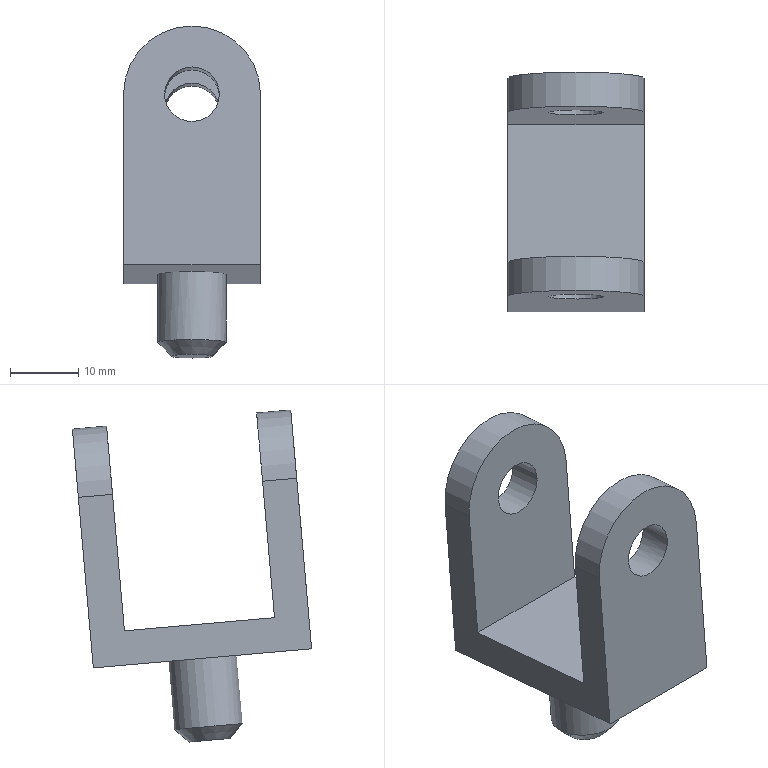Component | NX | LOCATING_SEAT | 1 solid | 15 faces | box 20 x 34.93 x 48.48 mm | volume 9156 mm3 | plane 9 | cylinder 5 | cone 1 | commonest cylinder face diameters 20 x2 8 x2 10 x1
STEP:
#1=CARTESIAN_POINT('',(0.,0.,0.));
#2=DIRECTION('',(0.,0.,1.));
#3=DIRECTION('',(1.,0.,0.));
#4=AXIS2_PLACEMENT_3D('',#1,#2,#3);
#5=CARTESIAN_POINT('',(285.941,457.133,-24.72));
#6=VERTEX_POINT('',#5);
#7=CARTESIAN_POINT('',(265.941,457.133,-24.72));
#8=VERTEX_POINT('',#7);
#9=CARTESIAN_POINT('',(275.941,457.133,-24.72));
#10=DIRECTION('',(0.,-0.9962,0.08716));
#11=DIRECTION('',(-1.,0.,0.));
#12=AXIS2_PLACEMENT_3D('',#9,#10,#11);
#13=CIRCLE('',#12,10.);
#14=CARTESIAN_POINT('',(275.941,462.114,-25.155));
#15=DIRECTION('',(0.,-0.9962,0.08716));
#16=DIRECTION('',(0.,0.08716,0.9962));
#17=AXIS2_PLACEMENT_3D('',#14,#15,#16);
#18=CYLINDRICAL_SURFACE('',#17,10.);
#19=CARTESIAN_POINT('',(-4.712,5.));
#20=DIRECTION('',(1.,0.));
#21=VECTOR('',#20,1.);
#22=LINE('',#19,#21);
#23=(GEOMETRIC_REPRESENTATION_CONTEXT(2)PARAMETRIC_REPRESENTATION_CONTEXT()REPRESENTATION_CONTEXT('',''));
#24=DEFINITIONAL_REPRESENTATION('',(#22),#23);
#25=PCURVE('',#18,#24);
#26=CARTESIAN_POINT('',(275.941,457.133,-24.72));
#27=DIRECTION('',(0.,-0.9962,0.08716));
#28=DIRECTION('',(0.,0.08716,0.9962));
#29=AXIS2_PLACEMENT_3D('',#26,#27,#28);
#30=PLANE('',#29);
#31=CARTESIAN_POINT('',(0.,0.));
#32=DIRECTION('',(0.,1.));
#33=AXIS2_PLACEMENT_2D('',#31,#32);
#34=CIRCLE('',#33,10.);
#35=(GEOMETRIC_REPRESENTATION_CONTEXT(2)PARAMETRIC_REPRESENTATION_CONTEXT()REPRESENTATION_CONTEXT('',''));
#36=DEFINITIONAL_REPRESENTATION('',(#34),#35);
#37=PCURVE('',#30,#36);
#38=SURFACE_CURVE('',#13,(#25,#37),.PCURVE_S1.);
#39=EDGE_CURVE('',#6,#8,#38,.T.);
#40=ORIENTED_EDGE('',*,*,#39,.F.);
#41=CARTESIAN_POINT('',(285.941,462.114,-25.155));
#42=VERTEX_POINT('',#41);
#43=CARTESIAN_POINT('',(285.941,462.114,-25.155));
#44=DIRECTION('',(0.,-0.9962,0.08716));
#45=VECTOR('',#44,1.);
#46=LINE('',#43,#45);
#47=CARTESIAN_POINT('',(-1.571,0.));
#48=DIRECTION('',(0.,1.));
#49=VECTOR('',#48,1.);
#50=LINE('',#47,#49);
#51=(GEOMETRIC_REPRESENTATION_CONTEXT(2)PARAMETRIC_REPRESENTATION_CONTEXT()REPRESENTATION_CONTEXT('',''));
#52=DEFINITIONAL_REPRESENTATION('',(#50),#51);
#53=PCURVE('',#18,#52);
#54=CARTESIAN_POINT('',(285.941,462.114,-25.155));
#55=DIRECTION('',(-1.,0.,0.));
#56=DIRECTION('',(0.,0.08716,0.9962));
#57=AXIS2_PLACEMENT_3D('',#54,#55,#56);
#58=PLANE('',#57);
#59=CARTESIAN_POINT('',(0.,0.));
#60=DIRECTION('',(-0.,-1.));
#61=VECTOR('',#60,1.);
#62=LINE('',#59,#61);
#63=(GEOMETRIC_REPRESENTATION_CONTEXT(2)PARAMETRIC_REPRESENTATION_CONTEXT()REPRESENTATION_CONTEXT('',''));
#64=DEFINITIONAL_REPRESENTATION('',(#62),#63);
#65=PCURVE('',#58,#64);
#66=SURFACE_CURVE('',#46,(#53,#65),.PCURVE_S1.);
#67=EDGE_CURVE('',#42,#6,#66,.T.);
#68=ORIENTED_EDGE('',*,*,#67,.F.);
#69=CARTESIAN_POINT('',(265.941,462.114,-25.155));
#70=VERTEX_POINT('',#69);
#71=CARTESIAN_POINT('',(275.941,462.114,-25.155));
#72=DIRECTION('',(0.,0.9962,-0.08716));
#73=DIRECTION('',(-1.,0.,0.));
#74=AXIS2_PLACEMENT_3D('',#71,#72,#73);
#75=CIRCLE('',#74,10.);
#76=CARTESIAN_POINT('',(1.571,0.));
#77=DIRECTION('',(-1.,0.));
#78=VECTOR('',#77,1.);
#79=LINE('',#76,#78);
#80=(GEOMETRIC_REPRESENTATION_CONTEXT(2)PARAMETRIC_REPRESENTATION_CONTEXT()REPRESENTATION_CONTEXT('',''));
#81=DEFINITIONAL_REPRESENTATION('',(#79),#80);
#82=PCURVE('',#18,#81);
#83=CARTESIAN_POINT('',(275.941,462.114,-25.155));
#84=DIRECTION('',(0.,0.9962,-0.08716));
#85=DIRECTION('',(0.,-0.08716,-0.9962));
#86=AXIS2_PLACEMENT_3D('',#83,#84,#85);
#87=PLANE('',#86);
#88=CARTESIAN_POINT('',(0.,0.));
#89=DIRECTION('',(0.,1.));
#90=AXIS2_PLACEMENT_2D('',#88,#89);
#91=CIRCLE('',#90,10.);
#92=(GEOMETRIC_REPRESENTATION_CONTEXT(2)PARAMETRIC_REPRESENTATION_CONTEXT()REPRESENTATION_CONTEXT('',''));
#93=DEFINITIONAL_REPRESENTATION('',(#91),#92);
#94=PCURVE('',#87,#93);
#95=SURFACE_CURVE('',#75,(#82,#94),.PCURVE_S1.);
#96=EDGE_CURVE('',#70,#42,#95,.T.);
#97=ORIENTED_EDGE('',*,*,#96,.F.);
#98=CARTESIAN_POINT('',(265.941,462.114,-25.155));
#99=DIRECTION('',(0.,-0.9962,0.08716));
#100=VECTOR('',#99,1.);
#101=LINE('',#98,#100);
#102=CARTESIAN_POINT('',(1.571,0.));
#103=DIRECTION('',(0.,1.));
#104=VECTOR('',#103,1.);
#105=LINE('',#102,#104);
#106=(GEOMETRIC_REPRESENTATION_CONTEXT(2)PARAMETRIC_REPRESENTATION_CONTEXT()REPRESENTATION_CONTEXT('',''));
#107=DEFINITIONAL_REPRESENTATION('',(#105),#106);
#108=PCURVE('',#18,#107);
#109=CARTESIAN_POINT('',(265.941,459.935,-50.06));
#110=DIRECTION('',(1.,-0.,-0.));
#111=DIRECTION('',(-0.,-0.08716,-0.9962));
#112=AXIS2_PLACEMENT_3D('',#109,#110,#111);
#113=PLANE('',#112);
#114=CARTESIAN_POINT('',(-25.,-0.));
#115=DIRECTION('',(0.,-1.));
#116=VECTOR('',#115,1.);
#117=LINE('',#114,#116);
#118=(GEOMETRIC_REPRESENTATION_CONTEXT(2)PARAMETRIC_REPRESENTATION_CONTEXT()REPRESENTATION_CONTEXT('',''));
#119=DEFINITIONAL_REPRESENTATION('',(#117),#118);
#120=PCURVE('',#113,#119);
#121=SURFACE_CURVE('',#101,(#108,#120),.PCURVE_S1.);
#122=EDGE_CURVE('',#70,#8,#121,.T.);
#123=ORIENTED_EDGE('',*,*,#122,.T.);
#124=EDGE_LOOP('',(#40,#68,#97,#123));
#125=FACE_BOUND('',#124,.T.);
#126=ADVANCED_FACE('',(#125),#18,.T.);
#127=CARTESIAN_POINT('',(285.941,455.39,-44.644));
#128=VERTEX_POINT('',#127);
#129=CARTESIAN_POINT('',(285.941,433.473,-42.726));
#130=VERTEX_POINT('',#129);
#131=CARTESIAN_POINT('',(285.941,455.39,-44.644));
#132=DIRECTION('',(0.,-0.9962,0.08716));
#133=VECTOR('',#132,1.);
#134=LINE('',#131,#133);
#135=CARTESIAN_POINT('',(-20.,-5.));
#136=DIRECTION('',(-0.,-1.));
#137=VECTOR('',#136,1.);
#138=LINE('',#135,#137);
#139=(GEOMETRIC_REPRESENTATION_CONTEXT(2)PARAMETRIC_REPRESENTATION_CONTEXT()REPRESENTATION_CONTEXT('',''));
#140=DEFINITIONAL_REPRESENTATION('',(#138),#139);
#141=PCURVE('',#58,#140);
#142=CARTESIAN_POINT('',(265.941,455.39,-44.644));
#143=DIRECTION('',(0.,-0.08716,-0.9962));
#144=DIRECTION('',(0.,-0.9962,0.08716));
#145=AXIS2_PLACEMENT_3D('',#142,#143,#144);
#146=PLANE('',#145);
#147=CARTESIAN_POINT('',(0.,-20.));
#148=DIRECTION('',(1.,0.));
#149=VECTOR('',#148,1.);
#150=LINE('',#147,#149);
#151=(GEOMETRIC_REPRESENTATION_CONTEXT(2)PARAMETRIC_REPRESENTATION_CONTEXT()REPRESENTATION_CONTEXT('',''));
#152=DEFINITIONAL_REPRESENTATION('',(#150),#151);
#153=PCURVE('',#146,#152);
#154=SURFACE_CURVE('',#134,(#141,#153),.PCURVE_S1.);
#155=EDGE_CURVE('',#128,#130,#154,.T.);
#156=ORIENTED_EDGE('',*,*,#155,.T.);
#157=CARTESIAN_POINT('',(285.941,435.216,-22.802));
#158=VERTEX_POINT('',#157);
#159=CARTESIAN_POINT('',(285.941,433.473,-42.726));
#160=DIRECTION('',(0.,0.08716,0.9962));
#161=VECTOR('',#160,1.);
#162=LINE('',#159,#161);
#163=CARTESIAN_POINT('',(-20.,-27.));
#164=DIRECTION('',(1.,0.));
#165=VECTOR('',#164,1.);
#166=LINE('',#163,#165);
#167=(GEOMETRIC_REPRESENTATION_CONTEXT(2)PARAMETRIC_REPRESENTATION_CONTEXT()REPRESENTATION_CONTEXT('',''));
#168=DEFINITIONAL_REPRESENTATION('',(#166),#167);
#169=PCURVE('',#58,#168);
#170=CARTESIAN_POINT('',(275.941,435.216,-22.802));
#171=DIRECTION('',(0.,-0.9962,0.08716));
#172=DIRECTION('',(0.,0.08716,0.9962));
#173=AXIS2_PLACEMENT_3D('',#170,#171,#172);
#174=PLANE('',#173);
#175=CARTESIAN_POINT('',(-20.,-10.));
#176=DIRECTION('',(1.,-0.));
#177=VECTOR('',#176,1.);
#178=LINE('',#175,#177);
#179=(GEOMETRIC_REPRESENTATION_CONTEXT(2)PARAMETRIC_REPRESENTATION_CONTEXT()REPRESENTATION_CONTEXT('',''));
#180=DEFINITIONAL_REPRESENTATION('',(#178),#179);
#181=PCURVE('',#174,#180);
#182=SURFACE_CURVE('',#162,(#169,#181),.PCURVE_S1.);
#183=EDGE_CURVE('',#130,#158,#182,.T.);
#184=ORIENTED_EDGE('',*,*,#183,.T.);
#185=CARTESIAN_POINT('',(285.941,430.235,-22.367));
#186=VERTEX_POINT('',#185);
#187=CARTESIAN_POINT('',(285.941,462.114,-25.155));
#188=DIRECTION('',(0.,-0.9962,0.08716));
#189=VECTOR('',#188,1.);
#190=LINE('',#187,#189);
#191=CARTESIAN_POINT('',(0.,0.));
#192=DIRECTION('',(-0.,-1.));
#193=VECTOR('',#192,1.);
#194=LINE('',#191,#193);
#195=(GEOMETRIC_REPRESENTATION_CONTEXT(2)PARAMETRIC_REPRESENTATION_CONTEXT()REPRESENTATION_CONTEXT('',''));
#196=DEFINITIONAL_REPRESENTATION('',(#194),#195);
#197=PCURVE('',#58,#196);
#198=CARTESIAN_POINT('',(275.941,462.114,-25.155));
#199=DIRECTION('',(0.,-0.9962,0.08716));
#200=DIRECTION('',(0.,0.08716,0.9962));
#201=AXIS2_PLACEMENT_3D('',#198,#199,#200);
#202=CYLINDRICAL_SURFACE('',#201,10.);
#203=CARTESIAN_POINT('',(4.712,0.));
#204=DIRECTION('',(0.,1.));
#205=VECTOR('',#204,1.);
#206=LINE('',#203,#205);
#207=(GEOMETRIC_REPRESENTATION_CONTEXT(2)PARAMETRIC_REPRESENTATION_CONTEXT()REPRESENTATION_CONTEXT('',''));
#208=DEFINITIONAL_REPRESENTATION('',(#206),#207);
#209=PCURVE('',#202,#208);
#210=SURFACE_CURVE('',#190,(#197,#209),.PCURVE_S1.);
#211=EDGE_CURVE('',#158,#186,#210,.T.);
#212=ORIENTED_EDGE('',*,*,#211,.T.);
#213=CARTESIAN_POINT('',(285.941,428.057,-47.271));
#214=VERTEX_POINT('',#213);
#215=CARTESIAN_POINT('',(285.941,430.235,-22.367));
#216=DIRECTION('',(-0.,-0.08716,-0.9962));
#217=VECTOR('',#216,1.);
#218=LINE('',#215,#217);
#219=CARTESIAN_POINT('',(0.,-32.));
#220=DIRECTION('',(-1.,0.));
#221=VECTOR('',#220,1.);
#222=LINE('',#219,#221);
#223=(GEOMETRIC_REPRESENTATION_CONTEXT(2)PARAMETRIC_REPRESENTATION_CONTEXT()REPRESENTATION_CONTEXT('',''));
#224=DEFINITIONAL_REPRESENTATION('',(#222),#223);
#225=PCURVE('',#58,#224);
#226=CARTESIAN_POINT('',(275.941,430.235,-22.367));
#227=DIRECTION('',(0.,0.9962,-0.08716));
#228=DIRECTION('',(0.,-0.08716,-0.9962));
#229=AXIS2_PLACEMENT_3D('',#226,#227,#228);
#230=PLANE('',#229);
#231=CARTESIAN_POINT('',(0.,-10.));
#232=DIRECTION('',(1.,0.));
#233=VECTOR('',#232,1.);
#234=LINE('',#231,#233);
#235=(GEOMETRIC_REPRESENTATION_CONTEXT(2)PARAMETRIC_REPRESENTATION_CONTEXT()REPRESENTATION_CONTEXT('',''));
#236=DEFINITIONAL_REPRESENTATION('',(#234),#235);
#237=PCURVE('',#230,#236);
#238=SURFACE_CURVE('',#218,(#225,#237),.PCURVE_S1.);
#239=EDGE_CURVE('',#186,#214,#238,.T.);
#240=ORIENTED_EDGE('',*,*,#239,.T.);
#241=CARTESIAN_POINT('',(285.941,459.935,-50.06));
#242=VERTEX_POINT('',#241);
#243=CARTESIAN_POINT('',(285.941,459.935,-50.06));
#244=DIRECTION('',(0.,-0.9962,0.08716));
#245=VECTOR('',#244,1.);
#246=LINE('',#243,#245);
#247=CARTESIAN_POINT('',(-25.,0.));
#248=DIRECTION('',(-0.,-1.));
#249=VECTOR('',#248,1.);
#250=LINE('',#247,#249);
#251=(GEOMETRIC_REPRESENTATION_CONTEXT(2)PARAMETRIC_REPRESENTATION_CONTEXT()REPRESENTATION_CONTEXT('',''));
#252=DEFINITIONAL_REPRESENTATION('',(#250),#251);
#253=PCURVE('',#58,#252);
#254=CARTESIAN_POINT('',(275.941,459.935,-50.06));
#255=DIRECTION('',(0.,0.08716,0.9962));
#256=DIRECTION('',(0.,0.9962,-0.08716));
#257=AXIS2_PLACEMENT_3D('',#254,#255,#256);
#258=PLANE('',#257);
#259=CARTESIAN_POINT('',(0.,-10.));
#260=DIRECTION('',(-1.,0.));
#261=VECTOR('',#260,1.);
#262=LINE('',#259,#261);
#263=(GEOMETRIC_REPRESENTATION_CONTEXT(2)PARAMETRIC_REPRESENTATION_CONTEXT()REPRESENTATION_CONTEXT('',''));
#264=DEFINITIONAL_REPRESENTATION('',(#262),#263);
#265=PCURVE('',#258,#264);
#266=SURFACE_CURVE('',#246,(#253,#265),.PCURVE_S1.);
#267=EDGE_CURVE('',#242,#214,#266,.T.);
#268=ORIENTED_EDGE('',*,*,#267,.F.);
#269=CARTESIAN_POINT('',(285.941,462.114,-25.155));
#270=DIRECTION('',(-0.,-0.08716,-0.9962));
#271=VECTOR('',#270,1.);
#272=LINE('',#269,#271);
#273=CARTESIAN_POINT('',(0.,0.));
#274=DIRECTION('',(-1.,0.));
#275=VECTOR('',#274,1.);
#276=LINE('',#273,#275);
#277=(GEOMETRIC_REPRESENTATION_CONTEXT(2)PARAMETRIC_REPRESENTATION_CONTEXT()REPRESENTATION_CONTEXT('',''));
#278=DEFINITIONAL_REPRESENTATION('',(#276),#277);
#279=PCURVE('',#58,#278);
#280=CARTESIAN_POINT('',(0.,-10.));
#281=DIRECTION('',(1.,0.));
#282=VECTOR('',#281,1.);
#283=LINE('',#280,#282);
#284=(GEOMETRIC_REPRESENTATION_CONTEXT(2)PARAMETRIC_REPRESENTATION_CONTEXT()REPRESENTATION_CONTEXT('',''));
#285=DEFINITIONAL_REPRESENTATION('',(#283),#284);
#286=PCURVE('',#87,#285);
#287=SURFACE_CURVE('',#272,(#279,#286),.PCURVE_S1.);
#288=EDGE_CURVE('',#42,#242,#287,.T.);
#289=ORIENTED_EDGE('',*,*,#288,.F.);
#290=ORIENTED_EDGE('',*,*,#67,.T.);
#291=CARTESIAN_POINT('',(285.941,455.39,-44.644));
#292=DIRECTION('',(0.,0.08716,0.9962));
#293=VECTOR('',#292,1.);
#294=LINE('',#291,#293);
#295=CARTESIAN_POINT('',(-20.,-5.));
#296=DIRECTION('',(1.,0.));
#297=VECTOR('',#296,1.);
#298=LINE('',#295,#297);
#299=(GEOMETRIC_REPRESENTATION_CONTEXT(2)PARAMETRIC_REPRESENTATION_CONTEXT()REPRESENTATION_CONTEXT('',''));
#300=DEFINITIONAL_REPRESENTATION('',(#298),#299);
#301=PCURVE('',#58,#300);
#302=CARTESIAN_POINT('',(-20.,-10.));
#303=DIRECTION('',(1.,-0.));
#304=VECTOR('',#303,1.);
#305=LINE('',#302,#304);
#306=(GEOMETRIC_REPRESENTATION_CONTEXT(2)PARAMETRIC_REPRESENTATION_CONTEXT()REPRESENTATION_CONTEXT('',''));
#307=DEFINITIONAL_REPRESENTATION('',(#305),#306);
#308=PCURVE('',#30,#307);
#309=SURFACE_CURVE('',#294,(#301,#308),.PCURVE_S1.);
#310=EDGE_CURVE('',#128,#6,#309,.T.);
#311=ORIENTED_EDGE('',*,*,#310,.F.);
#312=EDGE_LOOP('',(#156,#184,#212,#240,#268,#289,#290,#311));
#313=FACE_BOUND('',#312,.T.);
#314=ADVANCED_FACE('',(#313),#58,.F.);
#315=CARTESIAN_POINT('',(270.941,443.996,-48.666));
#316=VERTEX_POINT('',#315);
#317=CARTESIAN_POINT('',(275.941,443.996,-48.666));
#318=DIRECTION('',(0.,-0.08716,-0.9962));
#319=DIRECTION('',(-1.,0.,0.));
#320=AXIS2_PLACEMENT_3D('',#317,#318,#319);
#321=CIRCLE('',#320,5.);
#322=CARTESIAN_POINT('',(-16.,5.));
#323=CARTESIAN_POINT('',(-7.34,5.));
#324=CARTESIAN_POINT('',(-11.67,-2.5));
#325=CARTESIAN_POINT('',(-16.,-10.));
#326=CARTESIAN_POINT('',(-20.33,-2.5));
#327=CARTESIAN_POINT('',(-24.66,5.));
#328=CARTESIAN_POINT('',(-16.,5.));
#329=(BOUNDED_CURVE()B_SPLINE_CURVE(2,(#322,#323,#324,#325,#326,#327,#328),.UNSPECIFIED.,.T.,.F.)B_SPLINE_CURVE_WITH_KNOTS((1,2,2,2,2,1),(-2.094,0.,2.094,4.189,6.283,8.378),.UNSPECIFIED.)CURVE()GEOMETRIC_REPRESENTATION_ITEM()RATIONAL_B_SPLINE_CURVE((1.,0.5,1.,0.5,1.,0.5,1.))REPRESENTATION_ITEM(''));
#330=(GEOMETRIC_REPRESENTATION_CONTEXT(2)PARAMETRIC_REPRESENTATION_CONTEXT()REPRESENTATION_CONTEXT('',''));
#331=DEFINITIONAL_REPRESENTATION('',(#329),#330);
#332=PCURVE('',#258,#331);
#333=CARTESIAN_POINT('',(275.941,442.95,-60.62));
#334=DIRECTION('',(0.,0.08716,0.9962));
#335=DIRECTION('',(0.,0.9962,-0.08716));
#336=AXIS2_PLACEMENT_3D('',#333,#334,#335);
#337=CYLINDRICAL_SURFACE('',#336,5.);
#338=CARTESIAN_POINT('',(7.854,12.));
#339=DIRECTION('',(-1.,0.));
#340=VECTOR('',#339,1.);
#341=LINE('',#338,#340);
#342=(GEOMETRIC_REPRESENTATION_CONTEXT(2)PARAMETRIC_REPRESENTATION_CONTEXT()REPRESENTATION_CONTEXT('',''));
#343=DEFINITIONAL_REPRESENTATION('',(#341),#342);
#344=PCURVE('',#337,#343);
#345=SURFACE_CURVE('',#321,(#332,#344),.PCURVE_S1.);
#346=EDGE_CURVE('',#316,#316,#345,.T.);
#347=ORIENTED_EDGE('',*,*,#346,.F.);
#348=EDGE_LOOP('',(#347));
#349=FACE_BOUND('',#348,.T.);
#350=CARTESIAN_POINT('',(265.941,428.057,-47.271));
#351=VERTEX_POINT('',#350);
#352=CARTESIAN_POINT('',(275.941,428.057,-47.271));
#353=DIRECTION('',(-1.,0.,0.));
#354=VECTOR('',#353,1.);
#355=LINE('',#352,#354);
#356=CARTESIAN_POINT('',(-32.,0.));
#357=DIRECTION('',(0.,1.));
#358=VECTOR('',#357,1.);
#359=LINE('',#356,#358);
#360=(GEOMETRIC_REPRESENTATION_CONTEXT(2)PARAMETRIC_REPRESENTATION_CONTEXT()REPRESENTATION_CONTEXT('',''));
#361=DEFINITIONAL_REPRESENTATION('',(#359),#360);
#362=PCURVE('',#258,#361);
#363=CARTESIAN_POINT('',(25.,0.));
#364=DIRECTION('',(0.,1.));
#365=VECTOR('',#364,1.);
#366=LINE('',#363,#365);
#367=(GEOMETRIC_REPRESENTATION_CONTEXT(2)PARAMETRIC_REPRESENTATION_CONTEXT()REPRESENTATION_CONTEXT('',''));
#368=DEFINITIONAL_REPRESENTATION('',(#366),#367);
#369=PCURVE('',#230,#368);
#370=SURFACE_CURVE('',#355,(#362,#369),.PCURVE_S1.);
#371=EDGE_CURVE('',#214,#351,#370,.T.);
#372=ORIENTED_EDGE('',*,*,#371,.T.);
#373=CARTESIAN_POINT('',(265.941,459.935,-50.06));
#374=VERTEX_POINT('',#373);
#375=CARTESIAN_POINT('',(265.941,459.935,-50.06));
#376=DIRECTION('',(0.,-0.9962,0.08716));
#377=VECTOR('',#376,1.);
#378=LINE('',#375,#377);
#379=CARTESIAN_POINT('',(0.,10.));
#380=DIRECTION('',(-1.,0.));
#381=VECTOR('',#380,1.);
#382=LINE('',#379,#381);
#383=(GEOMETRIC_REPRESENTATION_CONTEXT(2)PARAMETRIC_REPRESENTATION_CONTEXT()REPRESENTATION_CONTEXT('',''));
#384=DEFINITIONAL_REPRESENTATION('',(#382),#383);
#385=PCURVE('',#258,#384);
#386=CARTESIAN_POINT('',(0.,0.));
#387=DIRECTION('',(0.,-1.));
#388=VECTOR('',#387,1.);
#389=LINE('',#386,#388);
#390=(GEOMETRIC_REPRESENTATION_CONTEXT(2)PARAMETRIC_REPRESENTATION_CONTEXT()REPRESENTATION_CONTEXT('',''));
#391=DEFINITIONAL_REPRESENTATION('',(#389),#390);
#392=PCURVE('',#113,#391);
#393=SURFACE_CURVE('',#378,(#385,#392),.PCURVE_S1.);
#394=EDGE_CURVE('',#374,#351,#393,.T.);
#395=ORIENTED_EDGE('',*,*,#394,.F.);
#396=CARTESIAN_POINT('',(285.941,459.935,-50.06));
#397=DIRECTION('',(-1.,0.,0.));
#398=VECTOR('',#397,1.);
#399=LINE('',#396,#398);
#400=CARTESIAN_POINT('',(0.,-10.));
#401=DIRECTION('',(0.,1.));
#402=VECTOR('',#401,1.);
#403=LINE('',#400,#402);
#404=(GEOMETRIC_REPRESENTATION_CONTEXT(2)PARAMETRIC_REPRESENTATION_CONTEXT()REPRESENTATION_CONTEXT('',''));
#405=DEFINITIONAL_REPRESENTATION('',(#403),#404);
#406=PCURVE('',#258,#405);
#407=CARTESIAN_POINT('',(25.,-10.));
#408=DIRECTION('',(0.,1.));
#409=VECTOR('',#408,1.);
#410=LINE('',#407,#409);
#411=(GEOMETRIC_REPRESENTATION_CONTEXT(2)PARAMETRIC_REPRESENTATION_CONTEXT()REPRESENTATION_CONTEXT('',''));
#412=DEFINITIONAL_REPRESENTATION('',(#410),#411);
#413=PCURVE('',#87,#412);
#414=SURFACE_CURVE('',#399,(#406,#413),.PCURVE_S1.);
#415=EDGE_CURVE('',#242,#374,#414,.T.);
#416=ORIENTED_EDGE('',*,*,#415,.F.);
#417=ORIENTED_EDGE('',*,*,#267,.T.);
#418=EDGE_LOOP('',(#372,#395,#416,#417));
#419=FACE_BOUND('',#418,.T.);
#420=ADVANCED_FACE('',(#349,#419),#258,.F.);
#421=CARTESIAN_POINT('',(265.941,435.216,-22.802));
#422=VERTEX_POINT('',#421);
#423=CARTESIAN_POINT('',(265.941,430.235,-22.367));
#424=VERTEX_POINT('',#423);
#425=CARTESIAN_POINT('',(265.941,462.114,-25.155));
#426=DIRECTION('',(0.,-0.9962,0.08716));
#427=VECTOR('',#426,1.);
#428=LINE('',#425,#427);
#429=CARTESIAN_POINT('',(-25.,-0.));
#430=DIRECTION('',(0.,-1.));
#431=VECTOR('',#430,1.);
#432=LINE('',#429,#431);
#433=(GEOMETRIC_REPRESENTATION_CONTEXT(2)PARAMETRIC_REPRESENTATION_CONTEXT()REPRESENTATION_CONTEXT('',''));
#434=DEFINITIONAL_REPRESENTATION('',(#432),#433);
#435=PCURVE('',#113,#434);
#436=CARTESIAN_POINT('',(7.854,0.));
#437=DIRECTION('',(0.,1.));
#438=VECTOR('',#437,1.);
#439=LINE('',#436,#438);
#440=(GEOMETRIC_REPRESENTATION_CONTEXT(2)PARAMETRIC_REPRESENTATION_CONTEXT()REPRESENTATION_CONTEXT('',''));
#441=DEFINITIONAL_REPRESENTATION('',(#439),#440);
#442=PCURVE('',#202,#441);
#443=SURFACE_CURVE('',#428,(#435,#442),.PCURVE_S1.);
#444=EDGE_CURVE('',#422,#424,#443,.T.);
#445=ORIENTED_EDGE('',*,*,#444,.F.);
#446=CARTESIAN_POINT('',(265.941,433.473,-42.726));
#447=VERTEX_POINT('',#446);
#448=CARTESIAN_POINT('',(265.941,435.216,-22.802));
#449=DIRECTION('',(-0.,-0.08716,-0.9962));
#450=VECTOR('',#449,1.);
#451=LINE('',#448,#450);
#452=CARTESIAN_POINT('',(-25.,-27.));
#453=DIRECTION('',(1.,0.));
#454=VECTOR('',#453,1.);
#455=LINE('',#452,#454);
#456=(GEOMETRIC_REPRESENTATION_CONTEXT(2)PARAMETRIC_REPRESENTATION_CONTEXT()REPRESENTATION_CONTEXT('',''));
#457=DEFINITIONAL_REPRESENTATION('',(#455),#456);
#458=PCURVE('',#113,#457);
#459=CARTESIAN_POINT('',(0.,10.));
#460=DIRECTION('',(-1.,0.));
#461=VECTOR('',#460,1.);
#462=LINE('',#459,#461);
#463=(GEOMETRIC_REPRESENTATION_CONTEXT(2)PARAMETRIC_REPRESENTATION_CONTEXT()REPRESENTATION_CONTEXT('',''));
#464=DEFINITIONAL_REPRESENTATION('',(#462),#463);
#465=PCURVE('',#174,#464);
#466=SURFACE_CURVE('',#451,(#458,#465),.PCURVE_S1.);
#467=EDGE_CURVE('',#422,#447,#466,.T.);
#468=ORIENTED_EDGE('',*,*,#467,.T.);
#469=CARTESIAN_POINT('',(265.941,455.39,-44.644));
#470=VERTEX_POINT('',#469);
#471=CARTESIAN_POINT('',(265.941,455.39,-44.644));
#472=DIRECTION('',(0.,-0.9962,0.08716));
#473=VECTOR('',#472,1.);
#474=LINE('',#471,#473);
#475=CARTESIAN_POINT('',(-5.,-5.));
#476=DIRECTION('',(0.,-1.));
#477=VECTOR('',#476,1.);
#478=LINE('',#475,#477);
#479=(GEOMETRIC_REPRESENTATION_CONTEXT(2)PARAMETRIC_REPRESENTATION_CONTEXT()REPRESENTATION_CONTEXT('',''));
#480=DEFINITIONAL_REPRESENTATION('',(#478),#479);
#481=PCURVE('',#113,#480);
#482=CARTESIAN_POINT('',(0.,0.));
#483=DIRECTION('',(1.,0.));
#484=VECTOR('',#483,1.);
#485=LINE('',#482,#484);
#486=(GEOMETRIC_REPRESENTATION_CONTEXT(2)PARAMETRIC_REPRESENTATION_CONTEXT()REPRESENTATION_CONTEXT('',''));
#487=DEFINITIONAL_REPRESENTATION('',(#485),#486);
#488=PCURVE('',#146,#487);
#489=SURFACE_CURVE('',#474,(#481,#488),.PCURVE_S1.);
#490=EDGE_CURVE('',#470,#447,#489,.T.);
#491=ORIENTED_EDGE('',*,*,#490,.F.);
#492=CARTESIAN_POINT('',(265.941,457.133,-24.72));
#493=DIRECTION('',(-0.,-0.08716,-0.9962));
#494=VECTOR('',#493,1.);
#495=LINE('',#492,#494);
#496=CARTESIAN_POINT('',(-25.,-5.));
#497=DIRECTION('',(1.,0.));
#498=VECTOR('',#497,1.);
#499=LINE('',#496,#498);
#500=(GEOMETRIC_REPRESENTATION_CONTEXT(2)PARAMETRIC_REPRESENTATION_CONTEXT()REPRESENTATION_CONTEXT('',''));
#501=DEFINITIONAL_REPRESENTATION('',(#499),#500);
#502=PCURVE('',#113,#501);
#503=CARTESIAN_POINT('',(0.,10.));
#504=DIRECTION('',(-1.,0.));
#505=VECTOR('',#504,1.);
#506=LINE('',#503,#505);
#507=(GEOMETRIC_REPRESENTATION_CONTEXT(2)PARAMETRIC_REPRESENTATION_CONTEXT()REPRESENTATION_CONTEXT('',''));
#508=DEFINITIONAL_REPRESENTATION('',(#506),#507);
#509=PCURVE('',#30,#508);
#510=SURFACE_CURVE('',#495,(#502,#509),.PCURVE_S1.);
#511=EDGE_CURVE('',#8,#470,#510,.T.);
#512=ORIENTED_EDGE('',*,*,#511,.F.);
#513=ORIENTED_EDGE('',*,*,#122,.F.);
#514=CARTESIAN_POINT('',(265.941,459.935,-50.06));
#515=DIRECTION('',(0.,0.08716,0.9962));
#516=VECTOR('',#515,1.);
#517=LINE('',#514,#516);
#518=CARTESIAN_POINT('',(0.,0.));
#519=DIRECTION('',(-1.,0.));
#520=VECTOR('',#519,1.);
#521=LINE('',#518,#520);
#522=(GEOMETRIC_REPRESENTATION_CONTEXT(2)PARAMETRIC_REPRESENTATION_CONTEXT()REPRESENTATION_CONTEXT('',''));
#523=DEFINITIONAL_REPRESENTATION('',(#521),#522);
#524=PCURVE('',#113,#523);
#525=CARTESIAN_POINT('',(25.,10.));
#526=DIRECTION('',(-1.,-0.));
#527=VECTOR('',#526,1.);
#528=LINE('',#525,#527);
#529=(GEOMETRIC_REPRESENTATION_CONTEXT(2)PARAMETRIC_REPRESENTATION_CONTEXT()REPRESENTATION_CONTEXT('',''));
#530=DEFINITIONAL_REPRESENTATION('',(#528),#529);
#531=PCURVE('',#87,#530);
#532=SURFACE_CURVE('',#517,(#524,#531),.PCURVE_S1.);
#533=EDGE_CURVE('',#374,#70,#532,.T.);
#534=ORIENTED_EDGE('',*,*,#533,.F.);
#535=ORIENTED_EDGE('',*,*,#394,.T.);
#536=CARTESIAN_POINT('',(265.941,428.057,-47.271));
#537=DIRECTION('',(0.,0.08716,0.9962));
#538=VECTOR('',#537,1.);
#539=LINE('',#536,#538);
#540=CARTESIAN_POINT('',(0.,-32.));
#541=DIRECTION('',(-1.,0.));
#542=VECTOR('',#541,1.);
#543=LINE('',#540,#542);
#544=(GEOMETRIC_REPRESENTATION_CONTEXT(2)PARAMETRIC_REPRESENTATION_CONTEXT()REPRESENTATION_CONTEXT('',''));
#545=DEFINITIONAL_REPRESENTATION('',(#543),#544);
#546=PCURVE('',#113,#545);
#547=CARTESIAN_POINT('',(25.,10.));
#548=DIRECTION('',(-1.,-0.));
#549=VECTOR('',#548,1.);
#550=LINE('',#547,#549);
#551=(GEOMETRIC_REPRESENTATION_CONTEXT(2)PARAMETRIC_REPRESENTATION_CONTEXT()REPRESENTATION_CONTEXT('',''));
#552=DEFINITIONAL_REPRESENTATION('',(#550),#551);
#553=PCURVE('',#230,#552);
#554=SURFACE_CURVE('',#539,(#546,#553),.PCURVE_S1.);
#555=EDGE_CURVE('',#351,#424,#554,.T.);
#556=ORIENTED_EDGE('',*,*,#555,.T.);
#557=EDGE_LOOP('',(#445,#468,#491,#512,#513,#534,#535,#556));
#558=FACE_BOUND('',#557,.T.);
#559=ADVANCED_FACE('',(#558),#113,.F.);
#560=ORIENTED_EDGE('',*,*,#211,.F.);
#561=CARTESIAN_POINT('',(275.941,435.216,-22.802));
#562=DIRECTION('',(0.,-0.9962,0.08716));
#563=DIRECTION('',(-1.,0.,0.));
#564=AXIS2_PLACEMENT_3D('',#561,#562,#563);
#565=CIRCLE('',#564,10.);
#566=CARTESIAN_POINT('',(1.571,27.));
#567=DIRECTION('',(1.,0.));
#568=VECTOR('',#567,1.);
#569=LINE('',#566,#568);
#570=(GEOMETRIC_REPRESENTATION_CONTEXT(2)PARAMETRIC_REPRESENTATION_CONTEXT()REPRESENTATION_CONTEXT('',''));
#571=DEFINITIONAL_REPRESENTATION('',(#569),#570);
#572=PCURVE('',#202,#571);
#573=CARTESIAN_POINT('',(0.,0.));
#574=DIRECTION('',(0.,1.));
#575=AXIS2_PLACEMENT_2D('',#573,#574);
#576=CIRCLE('',#575,10.);
#577=(GEOMETRIC_REPRESENTATION_CONTEXT(2)PARAMETRIC_REPRESENTATION_CONTEXT()REPRESENTATION_CONTEXT('',''));
#578=DEFINITIONAL_REPRESENTATION('',(#576),#577);
#579=PCURVE('',#174,#578);
#580=SURFACE_CURVE('',#565,(#572,#579),.PCURVE_S1.);
#581=EDGE_CURVE('',#158,#422,#580,.T.);
#582=ORIENTED_EDGE('',*,*,#581,.T.);
#583=ORIENTED_EDGE('',*,*,#444,.T.);
#584=CARTESIAN_POINT('',(275.941,430.235,-22.367));
#585=DIRECTION('',(0.,0.9962,-0.08716));
#586=DIRECTION('',(-1.,0.,0.));
#587=AXIS2_PLACEMENT_3D('',#584,#585,#586);
#588=CIRCLE('',#587,10.);
#589=CARTESIAN_POINT('',(7.854,32.));
#590=DIRECTION('',(-1.,0.));
#591=VECTOR('',#590,1.);
#592=LINE('',#589,#591);
#593=(GEOMETRIC_REPRESENTATION_CONTEXT(2)PARAMETRIC_REPRESENTATION_CONTEXT()REPRESENTATION_CONTEXT('',''));
#594=DEFINITIONAL_REPRESENTATION('',(#592),#593);
#595=PCURVE('',#202,#594);
#596=CARTESIAN_POINT('',(0.,0.));
#597=DIRECTION('',(0.,1.));
#598=AXIS2_PLACEMENT_2D('',#596,#597);
#599=CIRCLE('',#598,10.);
#600=(GEOMETRIC_REPRESENTATION_CONTEXT(2)PARAMETRIC_REPRESENTATION_CONTEXT()REPRESENTATION_CONTEXT('',''));
#601=DEFINITIONAL_REPRESENTATION('',(#599),#600);
#602=PCURVE('',#230,#601);
#603=SURFACE_CURVE('',#588,(#595,#602),.PCURVE_S1.);
#604=EDGE_CURVE('',#424,#186,#603,.T.);
#605=ORIENTED_EDGE('',*,*,#604,.T.);
#606=EDGE_LOOP('',(#560,#582,#583,#605));
#607=FACE_BOUND('',#606,.T.);
#608=ADVANCED_FACE('',(#607),#202,.T.);
#609=CARTESIAN_POINT('',(275.941,461.765,-29.14));
#610=VERTEX_POINT('',#609);
#611=CARTESIAN_POINT('',(275.941,462.462,-21.171));
#612=VERTEX_POINT('',#611);
#613=CARTESIAN_POINT('',(275.941,462.114,-25.155));
#614=DIRECTION('',(0.,0.9962,-0.08716));
#615=DIRECTION('',(0.,-0.08716,-0.9962));
#616=AXIS2_PLACEMENT_3D('',#613,#614,#615);
#617=CIRCLE('',#616,4.);
#618=CARTESIAN_POINT('',(0.,0.));
#619=DIRECTION('',(1.,0.));
#620=AXIS2_PLACEMENT_2D('',#618,#619);
#621=CIRCLE('',#620,4.);
#622=(GEOMETRIC_REPRESENTATION_CONTEXT(2)PARAMETRIC_REPRESENTATION_CONTEXT()REPRESENTATION_CONTEXT('',''));
#623=DEFINITIONAL_REPRESENTATION('',(#621),#622);
#624=PCURVE('',#87,#623);
#625=CARTESIAN_POINT('',(275.941,479.049,-26.637));
#626=DIRECTION('',(0.,-0.9962,0.08716));
#627=DIRECTION('',(0.,0.08716,0.9962));
#628=AXIS2_PLACEMENT_3D('',#625,#626,#627);
#629=CYLINDRICAL_SURFACE('',#628,4.);
#630=CARTESIAN_POINT('',(3.142,17.));
#631=DIRECTION('',(-1.,0.));
#632=VECTOR('',#631,1.);
#633=LINE('',#630,#632);
#634=(GEOMETRIC_REPRESENTATION_CONTEXT(2)PARAMETRIC_REPRESENTATION_CONTEXT()REPRESENTATION_CONTEXT('',''));
#635=DEFINITIONAL_REPRESENTATION('',(#633),#634);
#636=PCURVE('',#629,#635);
#637=SURFACE_CURVE('',#617,(#624,#636),.PCURVE_S1.);
#638=EDGE_CURVE('',#610,#612,#637,.T.);
#639=ORIENTED_EDGE('',*,*,#638,.F.);
#640=CARTESIAN_POINT('',(275.941,462.114,-25.155));
#641=DIRECTION('',(0.,0.9962,-0.08716));
#642=DIRECTION('',(0.,-0.08716,-0.9962));
#643=AXIS2_PLACEMENT_3D('',#640,#641,#642);
#644=CIRCLE('',#643,4.);
#645=CARTESIAN_POINT('',(0.,0.));
#646=DIRECTION('',(1.,0.));
#647=AXIS2_PLACEMENT_2D('',#645,#646);
#648=CIRCLE('',#647,4.);
#649=(GEOMETRIC_REPRESENTATION_CONTEXT(2)PARAMETRIC_REPRESENTATION_CONTEXT()REPRESENTATION_CONTEXT('',''));
#650=DEFINITIONAL_REPRESENTATION('',(#648),#649);
#651=PCURVE('',#87,#650);
#652=CARTESIAN_POINT('',(9.425,17.));
#653=DIRECTION('',(-1.,0.));
#654=VECTOR('',#653,1.);
#655=LINE('',#652,#654);
#656=(GEOMETRIC_REPRESENTATION_CONTEXT(2)PARAMETRIC_REPRESENTATION_CONTEXT()REPRESENTATION_CONTEXT('',''));
#657=DEFINITIONAL_REPRESENTATION('',(#655),#656);
#658=PCURVE('',#629,#657);
#659=SURFACE_CURVE('',#644,(#651,#658),.PCURVE_S1.);
#660=EDGE_CURVE('',#612,#610,#659,.T.);
#661=ORIENTED_EDGE('',*,*,#660,.F.);
#662=EDGE_LOOP('',(#639,#661));
#663=FACE_BOUND('',#662,.T.);
#664=ORIENTED_EDGE('',*,*,#288,.T.);
#665=ORIENTED_EDGE('',*,*,#415,.T.);
#666=ORIENTED_EDGE('',*,*,#533,.T.);
#667=ORIENTED_EDGE('',*,*,#96,.T.);
#668=EDGE_LOOP('',(#664,#665,#666,#667));
#669=FACE_BOUND('',#668,.T.);
#670=ADVANCED_FACE('',(#663,#669),#87,.T.);
#671=CARTESIAN_POINT('',(279.941,430.235,-22.367));
#672=VERTEX_POINT('',#671);
#673=CARTESIAN_POINT('',(275.941,430.584,-18.382));
#674=VERTEX_POINT('',#673);
#675=CARTESIAN_POINT('',(275.941,430.235,-22.367));
#676=DIRECTION('',(0.,-0.9962,0.08716));
#677=DIRECTION('',(1.,0.,0.));
#678=AXIS2_PLACEMENT_3D('',#675,#676,#677);
#679=CIRCLE('',#678,4.);
#680=CARTESIAN_POINT('',(0.,-4.));
#681=CARTESIAN_POINT('',(-6.928,-4.));
#682=CARTESIAN_POINT('',(-3.464,2.));
#683=CARTESIAN_POINT('',(-0.,8.));
#684=CARTESIAN_POINT('',(3.464,2.));
#685=CARTESIAN_POINT('',(6.928,-4.));
#686=CARTESIAN_POINT('',(0.,-4.));
#687=(BOUNDED_CURVE()B_SPLINE_CURVE(2,(#680,#681,#682,#683,#684,#685,#686),.UNSPECIFIED.,.T.,.F.)B_SPLINE_CURVE_WITH_KNOTS((1,2,2,2,2,1),(-2.094,0.,2.094,4.189,6.283,8.378),.UNSPECIFIED.)CURVE()GEOMETRIC_REPRESENTATION_ITEM()RATIONAL_B_SPLINE_CURVE((1.,0.5,1.,0.5,1.,0.5,1.))REPRESENTATION_ITEM(''));
#688=(GEOMETRIC_REPRESENTATION_CONTEXT(2)PARAMETRIC_REPRESENTATION_CONTEXT()REPRESENTATION_CONTEXT('',''));
#689=DEFINITIONAL_REPRESENTATION('',(#687),#688);
#690=PCURVE('',#230,#689);
#691=CARTESIAN_POINT('',(275.941,479.049,-26.637));
#692=DIRECTION('',(0.,-0.9962,0.08716));
#693=DIRECTION('',(0.,0.08716,0.9962));
#694=AXIS2_PLACEMENT_3D('',#691,#692,#693);
#695=CYLINDRICAL_SURFACE('',#694,4.);
#696=CARTESIAN_POINT('',(4.712,49.));
#697=DIRECTION('',(1.,0.));
#698=VECTOR('',#697,1.);
#699=LINE('',#696,#698);
#700=(GEOMETRIC_REPRESENTATION_CONTEXT(2)PARAMETRIC_REPRESENTATION_CONTEXT()REPRESENTATION_CONTEXT('',''));
#701=DEFINITIONAL_REPRESENTATION('',(#699),#700);
#702=PCURVE('',#695,#701);
#703=SURFACE_CURVE('',#679,(#690,#702),.PCURVE_S1.);
#704=EDGE_CURVE('',#672,#674,#703,.T.);
#705=ORIENTED_EDGE('',*,*,#704,.F.);
#706=CARTESIAN_POINT('',(275.941,430.235,-22.367));
#707=DIRECTION('',(0.,-0.9962,0.08716));
#708=DIRECTION('',(1.,0.,0.));
#709=AXIS2_PLACEMENT_3D('',#706,#707,#708);
#710=CIRCLE('',#709,4.);
#711=CARTESIAN_POINT('',(0.,-4.));
#712=CARTESIAN_POINT('',(-6.928,-4.));
#713=CARTESIAN_POINT('',(-3.464,2.));
#714=CARTESIAN_POINT('',(-0.,8.));
#715=CARTESIAN_POINT('',(3.464,2.));
#716=CARTESIAN_POINT('',(6.928,-4.));
#717=CARTESIAN_POINT('',(0.,-4.));
#718=(BOUNDED_CURVE()B_SPLINE_CURVE(2,(#711,#712,#713,#714,#715,#716,#717),.UNSPECIFIED.,.T.,.F.)B_SPLINE_CURVE_WITH_KNOTS((1,2,2,2,2,1),(-2.094,0.,2.094,4.189,6.283,8.378),.UNSPECIFIED.)CURVE()GEOMETRIC_REPRESENTATION_ITEM()RATIONAL_B_SPLINE_CURVE((1.,0.5,1.,0.5,1.,0.5,1.))REPRESENTATION_ITEM(''));
#719=(GEOMETRIC_REPRESENTATION_CONTEXT(2)PARAMETRIC_REPRESENTATION_CONTEXT()REPRESENTATION_CONTEXT('',''));
#720=DEFINITIONAL_REPRESENTATION('',(#718),#719);
#721=PCURVE('',#230,#720);
#722=CARTESIAN_POINT('',(-1.571,49.));
#723=DIRECTION('',(1.,0.));
#724=VECTOR('',#723,1.);
#725=LINE('',#722,#724);
#726=(GEOMETRIC_REPRESENTATION_CONTEXT(2)PARAMETRIC_REPRESENTATION_CONTEXT()REPRESENTATION_CONTEXT('',''));
#727=DEFINITIONAL_REPRESENTATION('',(#725),#726);
#728=PCURVE('',#695,#727);
#729=SURFACE_CURVE('',#710,(#721,#728),.PCURVE_S1.);
#730=EDGE_CURVE('',#674,#672,#729,.T.);
#731=ORIENTED_EDGE('',*,*,#730,.F.);
#732=EDGE_LOOP('',(#705,#731));
#733=FACE_BOUND('',#732,.T.);
#734=ORIENTED_EDGE('',*,*,#239,.F.);
#735=ORIENTED_EDGE('',*,*,#604,.F.);
#736=ORIENTED_EDGE('',*,*,#555,.F.);
#737=ORIENTED_EDGE('',*,*,#371,.F.);
#738=EDGE_LOOP('',(#734,#735,#736,#737));
#739=FACE_BOUND('',#738,.T.);
#740=ADVANCED_FACE('',(#733,#739),#230,.F.);
#741=CARTESIAN_POINT('',(275.941,438.143,-58.192));
#742=VERTEX_POINT('',#741);
#743=CARTESIAN_POINT('',(270.941,443.124,-58.628));
#744=VERTEX_POINT('',#743);
#745=CARTESIAN_POINT('',(275.941,443.124,-58.628));
#746=DIRECTION('',(0.,0.08716,0.9962));
#747=DIRECTION('',(0.,-0.9962,0.08716));
#748=AXIS2_PLACEMENT_3D('',#745,#746,#747);
#749=CIRCLE('',#748,5.);
#750=CARTESIAN_POINT('',(3.142,2.));
#751=DIRECTION('',(1.,0.));
#752=VECTOR('',#751,1.);
#753=LINE('',#750,#752);
#754=(GEOMETRIC_REPRESENTATION_CONTEXT(2)PARAMETRIC_REPRESENTATION_CONTEXT()REPRESENTATION_CONTEXT('',''));
#755=DEFINITIONAL_REPRESENTATION('',(#753),#754);
#756=PCURVE('',#337,#755);
#757=CARTESIAN_POINT('',(275.941,442.95,-60.62));
#758=DIRECTION('',(0.,0.08716,0.9962));
#759=DIRECTION('',(0.,0.9962,-0.08716));
#760=AXIS2_PLACEMENT_3D('',#757,#758,#759);
#761=CONICAL_SURFACE('',#760,3.,0.7854);
#762=CARTESIAN_POINT('',(3.142,2.));
#763=DIRECTION('',(1.,0.));
#764=VECTOR('',#763,1.);
#765=LINE('',#762,#764);
#766=(GEOMETRIC_REPRESENTATION_CONTEXT(2)PARAMETRIC_REPRESENTATION_CONTEXT()REPRESENTATION_CONTEXT('',''));
#767=DEFINITIONAL_REPRESENTATION('',(#765),#766);
#768=PCURVE('',#761,#767);
#769=SURFACE_CURVE('',#749,(#756,#768),.PCURVE_S1.);
#770=EDGE_CURVE('',#742,#744,#769,.T.);
#771=ORIENTED_EDGE('',*,*,#770,.T.);
#772=CARTESIAN_POINT('',(270.941,443.124,-58.628));
#773=CARTESIAN_POINT('',(270.941,443.996,-48.666));
#774=B_SPLINE_CURVE_WITH_KNOTS('',1,(#772,#773),.UNSPECIFIED.,.F.,.F.,(2,2),(2.,12.),.PIECEWISE_BEZIER_KNOTS.);
#775=CARTESIAN_POINT('',(7.854,0.));
#776=DIRECTION('',(0.,1.));
#777=VECTOR('',#776,1.);
#778=LINE('',#775,#777);
#779=(GEOMETRIC_REPRESENTATION_CONTEXT(2)PARAMETRIC_REPRESENTATION_CONTEXT()REPRESENTATION_CONTEXT('',''));
#780=DEFINITIONAL_REPRESENTATION('',(#778),#779);
#781=PCURVE('',#337,#780);
#782=CARTESIAN_POINT('',(1.571,0.));
#783=DIRECTION('',(0.,1.));
#784=VECTOR('',#783,1.);
#785=LINE('',#782,#784);
#786=(GEOMETRIC_REPRESENTATION_CONTEXT(2)PARAMETRIC_REPRESENTATION_CONTEXT()REPRESENTATION_CONTEXT('',''));
#787=DEFINITIONAL_REPRESENTATION('',(#785),#786);
#788=PCURVE('',#337,#787);
#789=SEAM_CURVE('',#774,(#781,#788),.PCURVE_S1.);
#790=EDGE_CURVE('',#744,#316,#789,.T.);
#791=ORIENTED_EDGE('',*,*,#790,.T.);
#792=ORIENTED_EDGE('',*,*,#346,.T.);
#793=ORIENTED_EDGE('',*,*,#790,.F.);
#794=CARTESIAN_POINT('',(275.941,443.124,-58.628));
#795=DIRECTION('',(0.,0.08716,0.9962));
#796=DIRECTION('',(0.,-0.9962,0.08716));
#797=AXIS2_PLACEMENT_3D('',#794,#795,#796);
#798=CIRCLE('',#797,5.);
#799=CARTESIAN_POINT('',(-3.142,2.));
#800=DIRECTION('',(1.,0.));
#801=VECTOR('',#800,1.);
#802=LINE('',#799,#801);
#803=(GEOMETRIC_REPRESENTATION_CONTEXT(2)PARAMETRIC_REPRESENTATION_CONTEXT()REPRESENTATION_CONTEXT('',''));
#804=DEFINITIONAL_REPRESENTATION('',(#802),#803);
#805=PCURVE('',#337,#804);
#806=CARTESIAN_POINT('',(3.142,2.));
#807=DIRECTION('',(1.,-0.));
#808=VECTOR('',#807,1.);
#809=LINE('',#806,#808);
#810=(GEOMETRIC_REPRESENTATION_CONTEXT(2)PARAMETRIC_REPRESENTATION_CONTEXT()REPRESENTATION_CONTEXT('',''));
#811=DEFINITIONAL_REPRESENTATION('',(#809),#810);
#812=PCURVE('',#761,#811);
#813=SURFACE_CURVE('',#798,(#805,#812),.PCURVE_S1.);
#814=EDGE_CURVE('',#744,#742,#813,.T.);
#815=ORIENTED_EDGE('',*,*,#814,.T.);
#816=EDGE_LOOP('',(#771,#791,#792,#793,#815));
#817=FACE_BOUND('',#816,.T.);
#818=ADVANCED_FACE('',(#817),#337,.T.);
#819=CARTESIAN_POINT('',(275.941,439.961,-60.359));
#820=VERTEX_POINT('',#819);
#821=CARTESIAN_POINT('',(275.941,442.95,-60.62));
#822=DIRECTION('',(0.,-0.08716,-0.9962));
#823=DIRECTION('',(0.,-0.9962,0.08716));
#824=AXIS2_PLACEMENT_3D('',#821,#822,#823);
#825=CIRCLE('',#824,3.);
#826=CARTESIAN_POINT('',(275.941,442.95,-60.62));
#827=DIRECTION('',(0.,-0.08716,-0.9962));
#828=DIRECTION('',(0.,-0.9962,0.08716));
#829=AXIS2_PLACEMENT_3D('',#826,#827,#828);
#830=PLANE('',#829);
#831=CARTESIAN_POINT('',(0.,0.));
#832=DIRECTION('',(1.,0.));
#833=AXIS2_PLACEMENT_2D('',#831,#832);
#834=CIRCLE('',#833,3.);
#835=(GEOMETRIC_REPRESENTATION_CONTEXT(2)PARAMETRIC_REPRESENTATION_CONTEXT()REPRESENTATION_CONTEXT('',''));
#836=DEFINITIONAL_REPRESENTATION('',(#834),#835);
#837=PCURVE('',#830,#836);
#838=CARTESIAN_POINT('',(9.425,-0.));
#839=DIRECTION('',(-1.,0.));
#840=VECTOR('',#839,1.);
#841=LINE('',#838,#840);
#842=(GEOMETRIC_REPRESENTATION_CONTEXT(2)PARAMETRIC_REPRESENTATION_CONTEXT()REPRESENTATION_CONTEXT('',''));
#843=DEFINITIONAL_REPRESENTATION('',(#841),#842);
#844=PCURVE('',#761,#843);
#845=SURFACE_CURVE('',#825,(#837,#844),.PCURVE_S1.);
#846=EDGE_CURVE('',#820,#820,#845,.T.);
#847=ORIENTED_EDGE('',*,*,#846,.T.);
#848=EDGE_LOOP('',(#847));
#849=FACE_BOUND('',#848,.T.);
#850=ADVANCED_FACE('',(#849),#830,.T.);
#851=ORIENTED_EDGE('',*,*,#770,.F.);
#852=CARTESIAN_POINT('',(275.941,439.961,-60.359));
#853=CARTESIAN_POINT('',(275.941,438.143,-58.192));
#854=B_SPLINE_CURVE_WITH_KNOTS('',1,(#852,#853),.UNSPECIFIED.,.F.,.F.,(2,2),(-0.,2.828),.PIECEWISE_BEZIER_KNOTS.);
#855=CARTESIAN_POINT('',(3.142,0.));
#856=DIRECTION('',(0.,1.));
#857=VECTOR('',#856,1.);
#858=LINE('',#855,#857);
#859=(GEOMETRIC_REPRESENTATION_CONTEXT(2)PARAMETRIC_REPRESENTATION_CONTEXT()REPRESENTATION_CONTEXT('',''));
#860=DEFINITIONAL_REPRESENTATION('',(#858),#859);
#861=PCURVE('',#761,#860);
#862=CARTESIAN_POINT('',(9.425,0.));
#863=DIRECTION('',(0.,1.));
#864=VECTOR('',#863,1.);
#865=LINE('',#862,#864);
#866=(GEOMETRIC_REPRESENTATION_CONTEXT(2)PARAMETRIC_REPRESENTATION_CONTEXT()REPRESENTATION_CONTEXT('',''));
#867=DEFINITIONAL_REPRESENTATION('',(#865),#866);
#868=PCURVE('',#761,#867);
#869=SEAM_CURVE('',#854,(#861,#868),.PCURVE_S1.);
#870=EDGE_CURVE('',#820,#742,#869,.T.);
#871=ORIENTED_EDGE('',*,*,#870,.F.);
#872=ORIENTED_EDGE('',*,*,#846,.F.);
#873=ORIENTED_EDGE('',*,*,#870,.T.);
#874=ORIENTED_EDGE('',*,*,#814,.F.);
#875=EDGE_LOOP('',(#851,#871,#872,#873,#874));
#876=FACE_BOUND('',#875,.T.);
#877=ADVANCED_FACE('',(#876),#761,.T.);
#878=CARTESIAN_POINT('',(265.941,433.473,-42.726));
#879=DIRECTION('',(-1.,0.,0.));
#880=VECTOR('',#879,1.);
#881=LINE('',#878,#880);
#882=CARTESIAN_POINT('',(22.,0.));
#883=DIRECTION('',(0.,1.));
#884=VECTOR('',#883,1.);
#885=LINE('',#882,#884);
#886=(GEOMETRIC_REPRESENTATION_CONTEXT(2)PARAMETRIC_REPRESENTATION_CONTEXT()REPRESENTATION_CONTEXT('',''));
#887=DEFINITIONAL_REPRESENTATION('',(#885),#886);
#888=PCURVE('',#146,#887);
#889=CARTESIAN_POINT('',(-20.,10.));
#890=DIRECTION('',(0.,1.));
#891=VECTOR('',#890,1.);
#892=LINE('',#889,#891);
#893=(GEOMETRIC_REPRESENTATION_CONTEXT(2)PARAMETRIC_REPRESENTATION_CONTEXT()REPRESENTATION_CONTEXT('',''));
#894=DEFINITIONAL_REPRESENTATION('',(#892),#893);
#895=PCURVE('',#174,#894);
#896=SURFACE_CURVE('',#881,(#888,#895),.PCURVE_S1.);
#897=EDGE_CURVE('',#130,#447,#896,.T.);
#898=ORIENTED_EDGE('',*,*,#897,.F.);
#899=ORIENTED_EDGE('',*,*,#155,.F.);
#900=CARTESIAN_POINT('',(265.941,455.39,-44.644));
#901=DIRECTION('',(-1.,0.,0.));
#902=VECTOR('',#901,1.);
#903=LINE('',#900,#902);
#904=CARTESIAN_POINT('',(0.,0.));
#905=DIRECTION('',(0.,1.));
#906=VECTOR('',#905,1.);
#907=LINE('',#904,#906);
#908=(GEOMETRIC_REPRESENTATION_CONTEXT(2)PARAMETRIC_REPRESENTATION_CONTEXT()REPRESENTATION_CONTEXT('',''));
#909=DEFINITIONAL_REPRESENTATION('',(#907),#908);
#910=PCURVE('',#146,#909);
#911=CARTESIAN_POINT('',(-20.,10.));
#912=DIRECTION('',(0.,1.));
#913=VECTOR('',#912,1.);
#914=LINE('',#911,#913);
#915=(GEOMETRIC_REPRESENTATION_CONTEXT(2)PARAMETRIC_REPRESENTATION_CONTEXT()REPRESENTATION_CONTEXT('',''));
#916=DEFINITIONAL_REPRESENTATION('',(#914),#915);
#917=PCURVE('',#30,#916);
#918=SURFACE_CURVE('',#903,(#910,#917),.PCURVE_S1.);
#919=EDGE_CURVE('',#128,#470,#918,.T.);
#920=ORIENTED_EDGE('',*,*,#919,.T.);
#921=ORIENTED_EDGE('',*,*,#490,.T.);
#922=EDGE_LOOP('',(#898,#899,#920,#921));
#923=FACE_BOUND('',#922,.T.);
#924=ADVANCED_FACE('',(#923),#146,.F.);
#925=CARTESIAN_POINT('',(275.941,457.481,-20.735));
#926=VERTEX_POINT('',#925);
#927=CARTESIAN_POINT('',(275.941,457.133,-24.72));
#928=DIRECTION('',(0.,-0.9962,0.08716));
#929=DIRECTION('',(0.,0.08716,0.9962));
#930=AXIS2_PLACEMENT_3D('',#927,#928,#929);
#931=CIRCLE('',#930,4.);
#932=CARTESIAN_POINT('',(0.,0.));
#933=DIRECTION('',(1.,0.));
#934=AXIS2_PLACEMENT_2D('',#932,#933);
#935=CIRCLE('',#934,4.);
#936=(GEOMETRIC_REPRESENTATION_CONTEXT(2)PARAMETRIC_REPRESENTATION_CONTEXT()REPRESENTATION_CONTEXT('',''));
#937=DEFINITIONAL_REPRESENTATION('',(#935),#936);
#938=PCURVE('',#30,#937);
#939=CARTESIAN_POINT('',(0.,22.));
#940=DIRECTION('',(1.,0.));
#941=VECTOR('',#940,1.);
#942=LINE('',#939,#941);
#943=(GEOMETRIC_REPRESENTATION_CONTEXT(2)PARAMETRIC_REPRESENTATION_CONTEXT()REPRESENTATION_CONTEXT('',''));
#944=DEFINITIONAL_REPRESENTATION('',(#942),#943);
#945=PCURVE('',#629,#944);
#946=SURFACE_CURVE('',#931,(#938,#945),.PCURVE_S1.);
#947=EDGE_CURVE('',#926,#926,#946,.T.);
#948=ORIENTED_EDGE('',*,*,#947,.F.);
#949=EDGE_LOOP('',(#948));
#950=FACE_BOUND('',#949,.T.);
#951=ORIENTED_EDGE('',*,*,#310,.T.);
#952=ORIENTED_EDGE('',*,*,#39,.T.);
#953=ORIENTED_EDGE('',*,*,#511,.T.);
#954=ORIENTED_EDGE('',*,*,#919,.F.);
#955=EDGE_LOOP('',(#951,#952,#953,#954));
#956=FACE_BOUND('',#955,.T.);
#957=ADVANCED_FACE('',(#950,#956),#30,.T.);
#958=CARTESIAN_POINT('',(275.941,435.565,-18.818));
#959=VERTEX_POINT('',#958);
#960=CARTESIAN_POINT('',(275.941,435.216,-22.802));
#961=DIRECTION('',(0.,-0.9962,0.08716));
#962=DIRECTION('',(0.,0.08716,0.9962));
#963=AXIS2_PLACEMENT_3D('',#960,#961,#962);
#964=CIRCLE('',#963,4.);
#965=CARTESIAN_POINT('',(0.,0.));
#966=DIRECTION('',(1.,0.));
#967=AXIS2_PLACEMENT_2D('',#965,#966);
#968=CIRCLE('',#967,4.);
#969=(GEOMETRIC_REPRESENTATION_CONTEXT(2)PARAMETRIC_REPRESENTATION_CONTEXT()REPRESENTATION_CONTEXT('',''));
#970=DEFINITIONAL_REPRESENTATION('',(#968),#969);
#971=PCURVE('',#174,#970);
#972=CARTESIAN_POINT('',(0.,44.));
#973=DIRECTION('',(1.,0.));
#974=VECTOR('',#973,1.);
#975=LINE('',#972,#974);
#976=(GEOMETRIC_REPRESENTATION_CONTEXT(2)PARAMETRIC_REPRESENTATION_CONTEXT()REPRESENTATION_CONTEXT('',''));
#977=DEFINITIONAL_REPRESENTATION('',(#975),#976);
#978=PCURVE('',#695,#977);
#979=SURFACE_CURVE('',#964,(#971,#978),.PCURVE_S1.);
#980=EDGE_CURVE('',#959,#959,#979,.T.);
#981=ORIENTED_EDGE('',*,*,#980,.T.);
#982=EDGE_LOOP('',(#981));
#983=FACE_BOUND('',#982,.T.);
#984=ORIENTED_EDGE('',*,*,#183,.F.);
#985=ORIENTED_EDGE('',*,*,#897,.T.);
#986=ORIENTED_EDGE('',*,*,#467,.F.);
#987=ORIENTED_EDGE('',*,*,#581,.F.);
#988=EDGE_LOOP('',(#984,#985,#986,#987));
#989=FACE_BOUND('',#988,.T.);
#990=ADVANCED_FACE('',(#983,#989),#174,.F.);
#991=ORIENTED_EDGE('',*,*,#730,.F.);
#992=CARTESIAN_POINT('',(275.941,435.565,-18.818));
#993=CARTESIAN_POINT('',(275.941,430.584,-18.382));
#994=B_SPLINE_CURVE_WITH_KNOTS('',1,(#992,#993),.UNSPECIFIED.,.F.,.F.,(2,2),(44.,49.),.PIECEWISE_BEZIER_KNOTS.);
#995=CARTESIAN_POINT('',(0.,0.));
#996=DIRECTION('',(0.,1.));
#997=VECTOR('',#996,1.);
#998=LINE('',#995,#997);
#999=(GEOMETRIC_REPRESENTATION_CONTEXT(2)PARAMETRIC_REPRESENTATION_CONTEXT()REPRESENTATION_CONTEXT('',''));
#1000=DEFINITIONAL_REPRESENTATION('',(#998),#999);
#1001=PCURVE('',#695,#1000);
#1002=CARTESIAN_POINT('',(6.283,0.));
#1003=DIRECTION('',(0.,1.));
#1004=VECTOR('',#1003,1.);
#1005=LINE('',#1002,#1004);
#1006=(GEOMETRIC_REPRESENTATION_CONTEXT(2)PARAMETRIC_REPRESENTATION_CONTEXT()REPRESENTATION_CONTEXT('',''));
#1007=DEFINITIONAL_REPRESENTATION('',(#1005),#1006);
#1008=PCURVE('',#695,#1007);
#1009=SEAM_CURVE('',#994,(#1001,#1008),.PCURVE_S1.);
#1010=EDGE_CURVE('',#959,#674,#1009,.T.);
#1011=ORIENTED_EDGE('',*,*,#1010,.F.);
#1012=ORIENTED_EDGE('',*,*,#980,.T.);
#1013=ORIENTED_EDGE('',*,*,#1010,.T.);
#1014=ORIENTED_EDGE('',*,*,#704,.F.);
#1015=EDGE_LOOP('',(#991,#1011,#1012,#1013,#1014));
#1016=FACE_BOUND('',#1015,.F.);
#1017=ADVANCED_FACE('',(#1016),#695,.F.);
#1018=ORIENTED_EDGE('',*,*,#660,.F.);
#1019=CARTESIAN_POINT('',(275.941,462.462,-21.171));
#1020=CARTESIAN_POINT('',(275.941,457.481,-20.735));
#1021=B_SPLINE_CURVE_WITH_KNOTS('',1,(#1019,#1020),.UNSPECIFIED.,.F.,.F.,(2,2),(17.,22.),.PIECEWISE_BEZIER_KNOTS.);
#1022=CARTESIAN_POINT('',(6.283,0.));
#1023=DIRECTION('',(0.,1.));
#1024=VECTOR('',#1023,1.);
#1025=LINE('',#1022,#1024);
#1026=(GEOMETRIC_REPRESENTATION_CONTEXT(2)PARAMETRIC_REPRESENTATION_CONTEXT()REPRESENTATION_CONTEXT('',''));
#1027=DEFINITIONAL_REPRESENTATION('',(#1025),#1026);
#1028=PCURVE('',#629,#1027);
#1029=CARTESIAN_POINT('',(0.,0.));
#1030=DIRECTION('',(0.,1.));
#1031=VECTOR('',#1030,1.);
#1032=LINE('',#1029,#1031);
#1033=(GEOMETRIC_REPRESENTATION_CONTEXT(2)PARAMETRIC_REPRESENTATION_CONTEXT()REPRESENTATION_CONTEXT('',''));
#1034=DEFINITIONAL_REPRESENTATION('',(#1032),#1033);
#1035=PCURVE('',#629,#1034);
#1036=SEAM_CURVE('',#1021,(#1028,#1035),.PCURVE_S1.);
#1037=EDGE_CURVE('',#612,#926,#1036,.T.);
#1038=ORIENTED_EDGE('',*,*,#1037,.T.);
#1039=ORIENTED_EDGE('',*,*,#947,.F.);
#1040=ORIENTED_EDGE('',*,*,#1037,.F.);
#1041=ORIENTED_EDGE('',*,*,#638,.F.);
#1042=EDGE_LOOP('',(#1018,#1038,#1039,#1040,#1041));
#1043=FACE_BOUND('',#1042,.F.);
#1044=ADVANCED_FACE('',(#1043),#629,.F.);
#1045=CLOSED_SHELL('',(#126,#314,#420,#559,#608,#670,#740,#818,#850,#877,#924,#957,#990,#1017,#1044));
#1046=MANIFOLD_SOLID_BREP('',#1045);
#1047=(LENGTH_UNIT()NAMED_UNIT(*)SI_UNIT(.MILLI.,.METRE.));
#1048=UNCERTAINTY_MEASURE_WITH_UNIT(LENGTH_MEASURE(0.000002),#1047,'','');
#1049=(NAMED_UNIT(*)PLANE_ANGLE_UNIT()SI_UNIT($,.RADIAN.));
#1050=(NAMED_UNIT(*)SI_UNIT($,.STERADIAN.)SOLID_ANGLE_UNIT());
#1051=(GEOMETRIC_REPRESENTATION_CONTEXT(3)GLOBAL_UNCERTAINTY_ASSIGNED_CONTEXT((#1048))GLOBAL_UNIT_ASSIGNED_CONTEXT((#1047,#1049,#1050))REPRESENTATION_CONTEXT('',''));
#1052=ADVANCED_BREP_SHAPE_REPRESENTATION('',(#4,#1046),#1051);